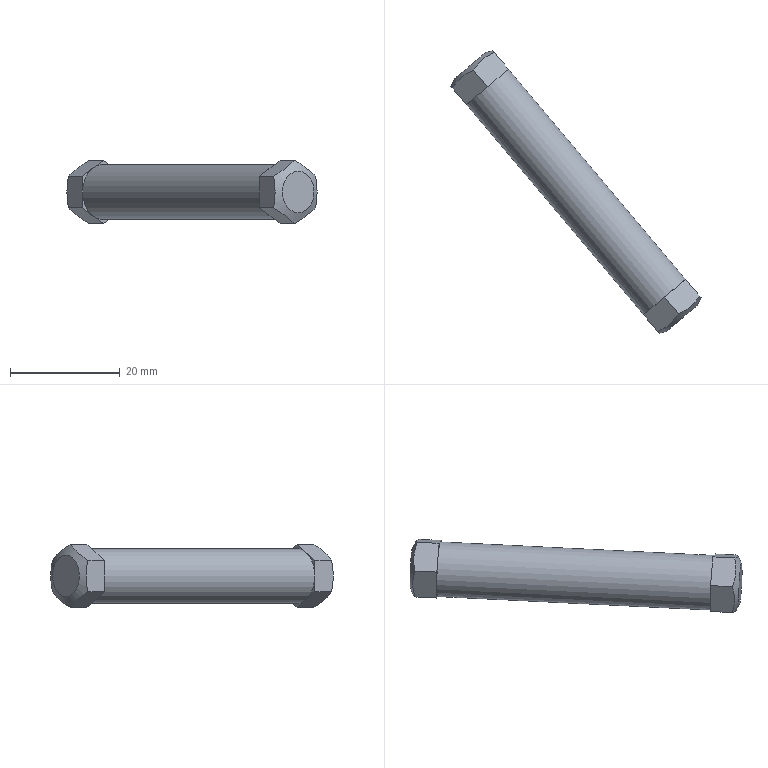Component | NX | PERNO | 1 solid | 29 faces | volume 4760 mm3 | plane 26 | cone 2 | cylinder 1 | commonest cylinder face diameters 10 x1